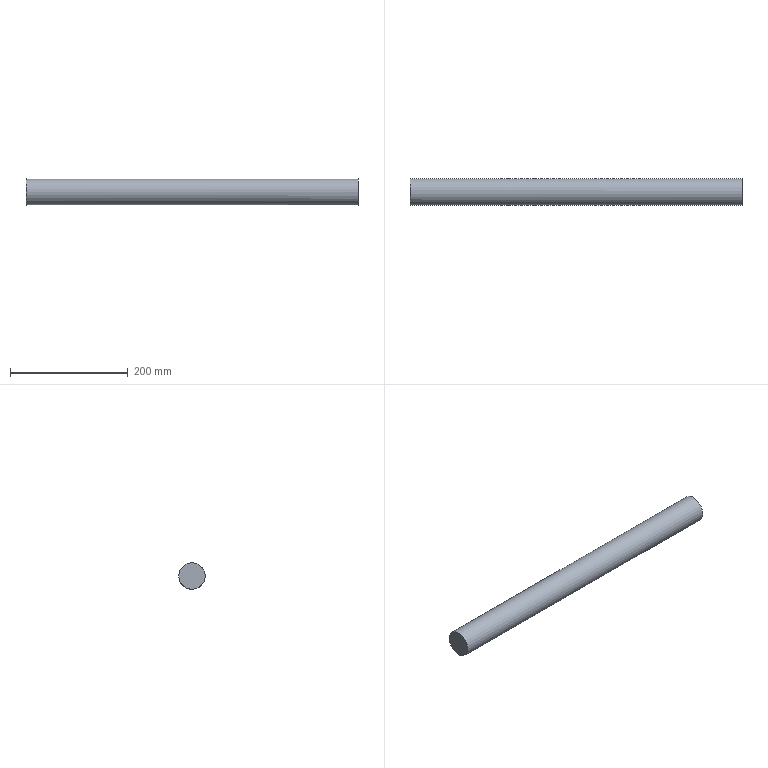Component | NX | DRIVEN_SHAFT | 1 solid | 12 faces | volume 895275 mm3 | plane 8 | cylinder 4 | commonest cylinder face diameters 8 x2 45 x1 14 x1